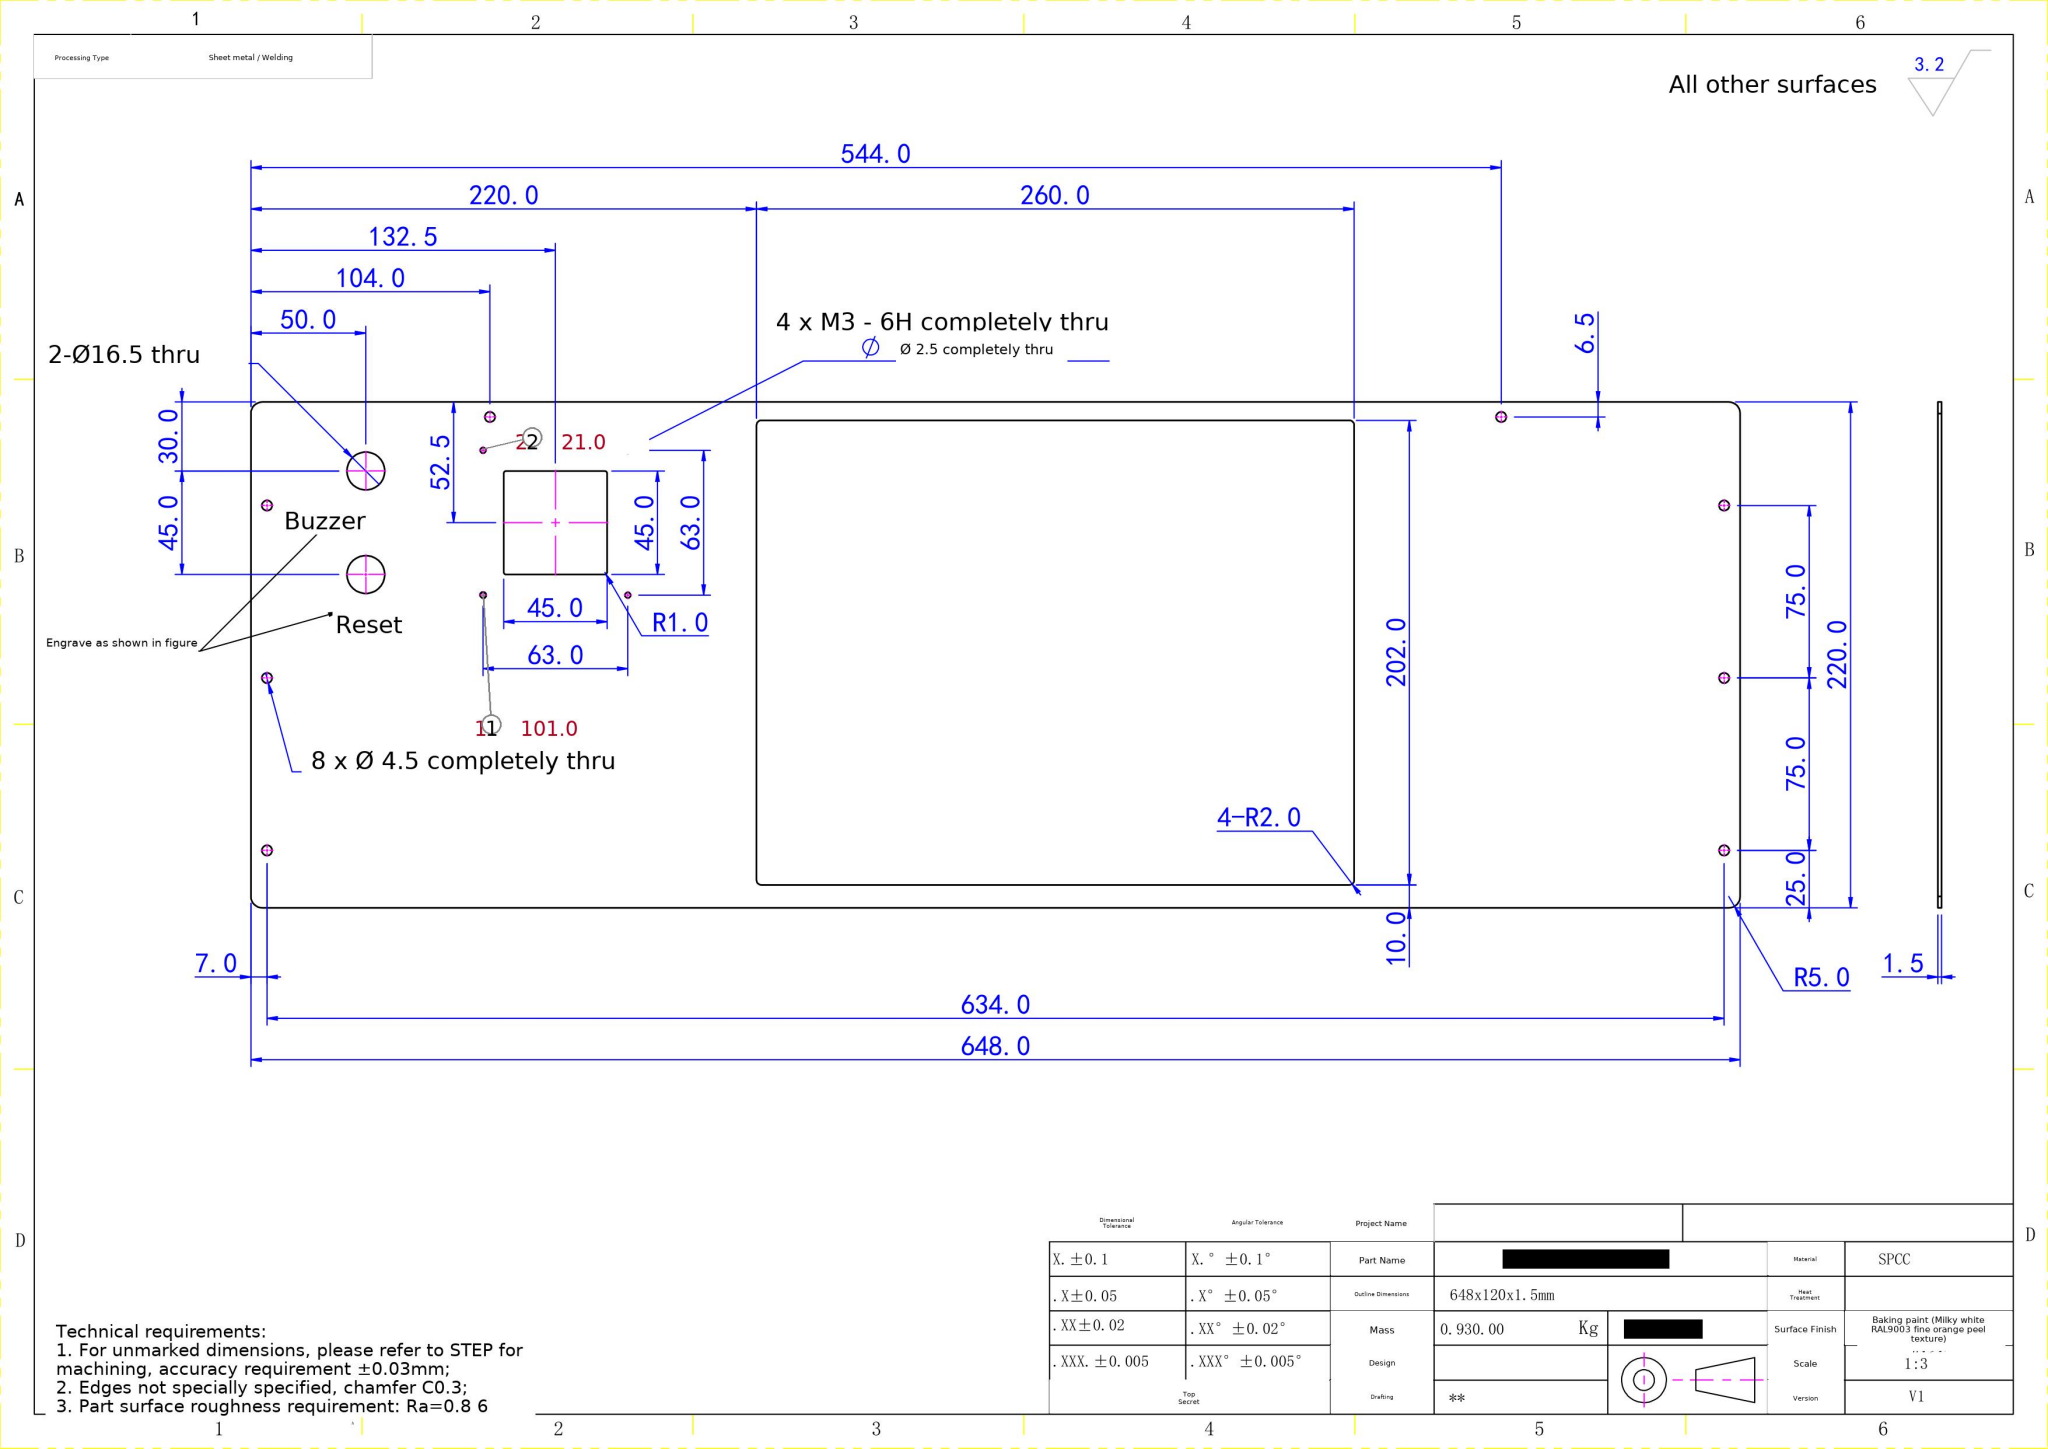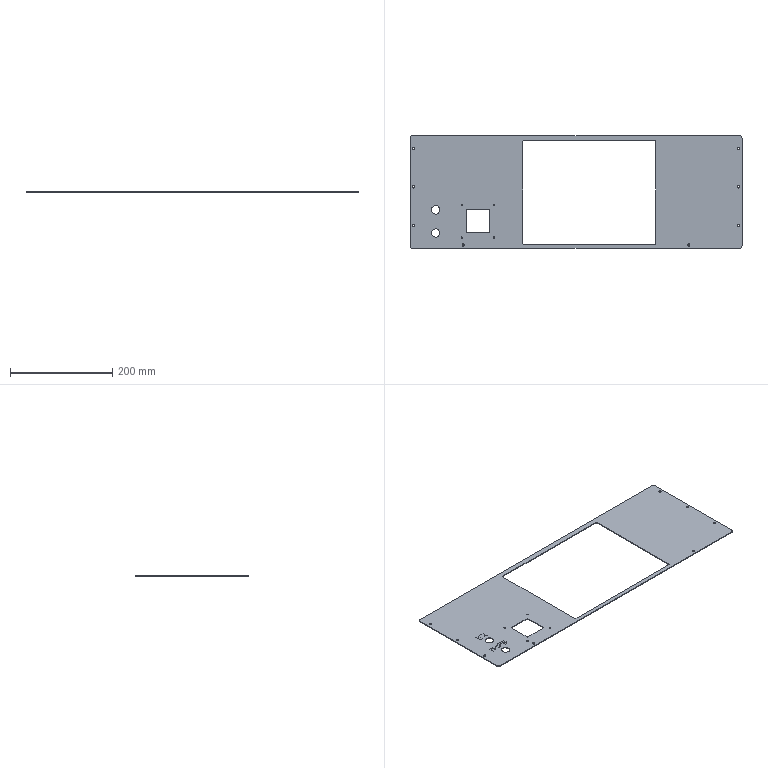Part | SolidWorks | mm | material SPCC | 1 solid | 412 faces | box 648 x 220 x 1.5 mm | volume 131133 mm3 | plane 277 | spline 95 | cylinder 40 | commonest cylinder face diameters 4.5 x16 2.5 x8 16.5 x4 10 x4 2 x4 4 x4